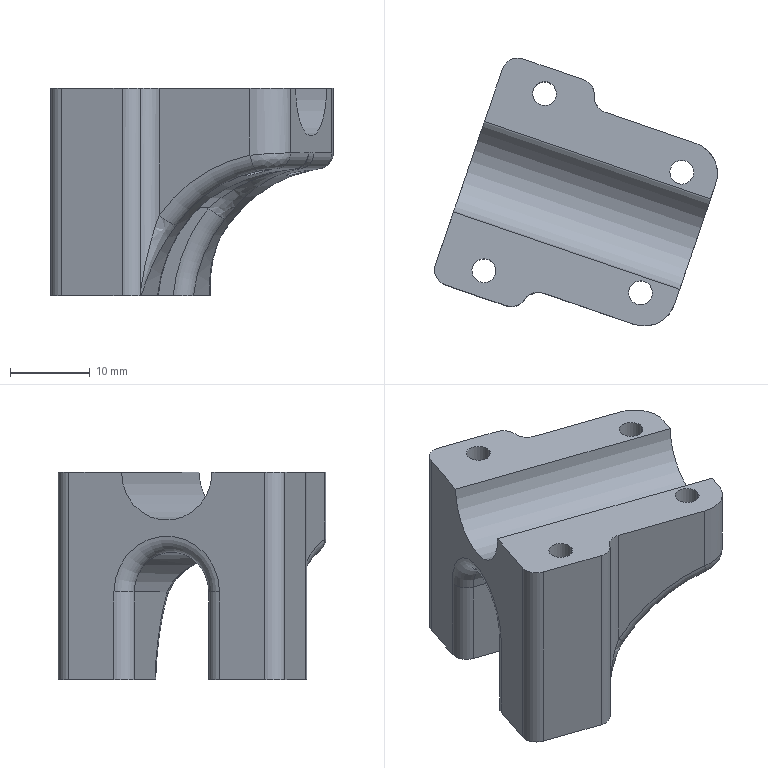Component | SolidWorks | UpperAndLowerPlateLowerConnectionPart-1 | 1 solid | 50 faces | volume 10529 mm3 | cylinder 24 | plane 12 | spline 6 | torus 6 | sphere 2 | commonest cylinder face diameters 4 x10 3 x8 8 x2 36 x2 10 x1 12 x1